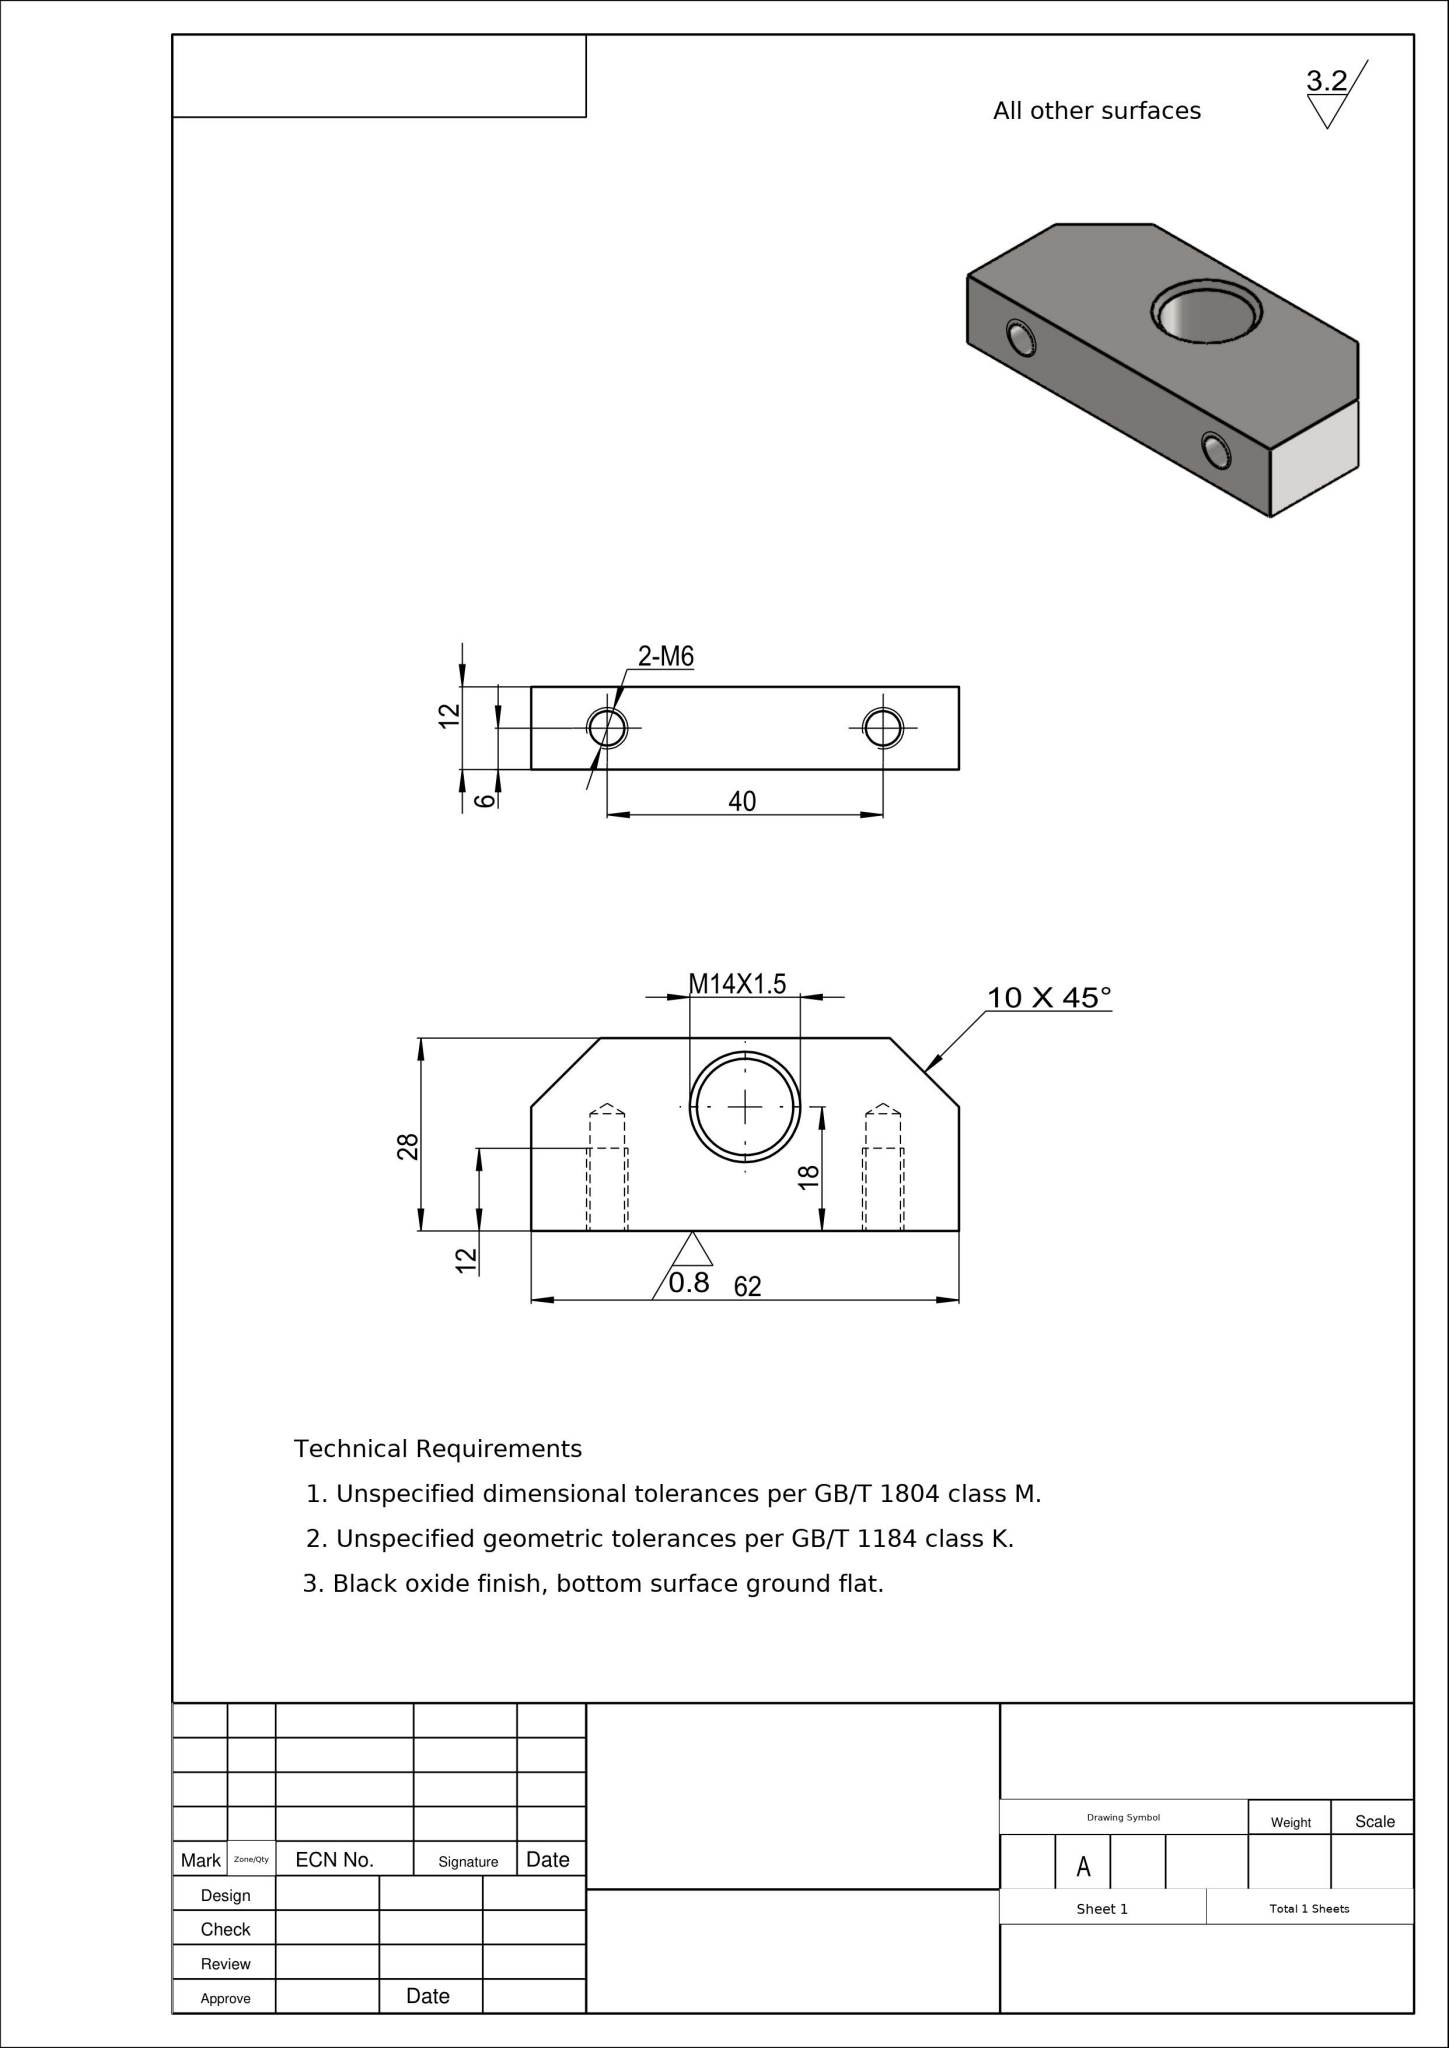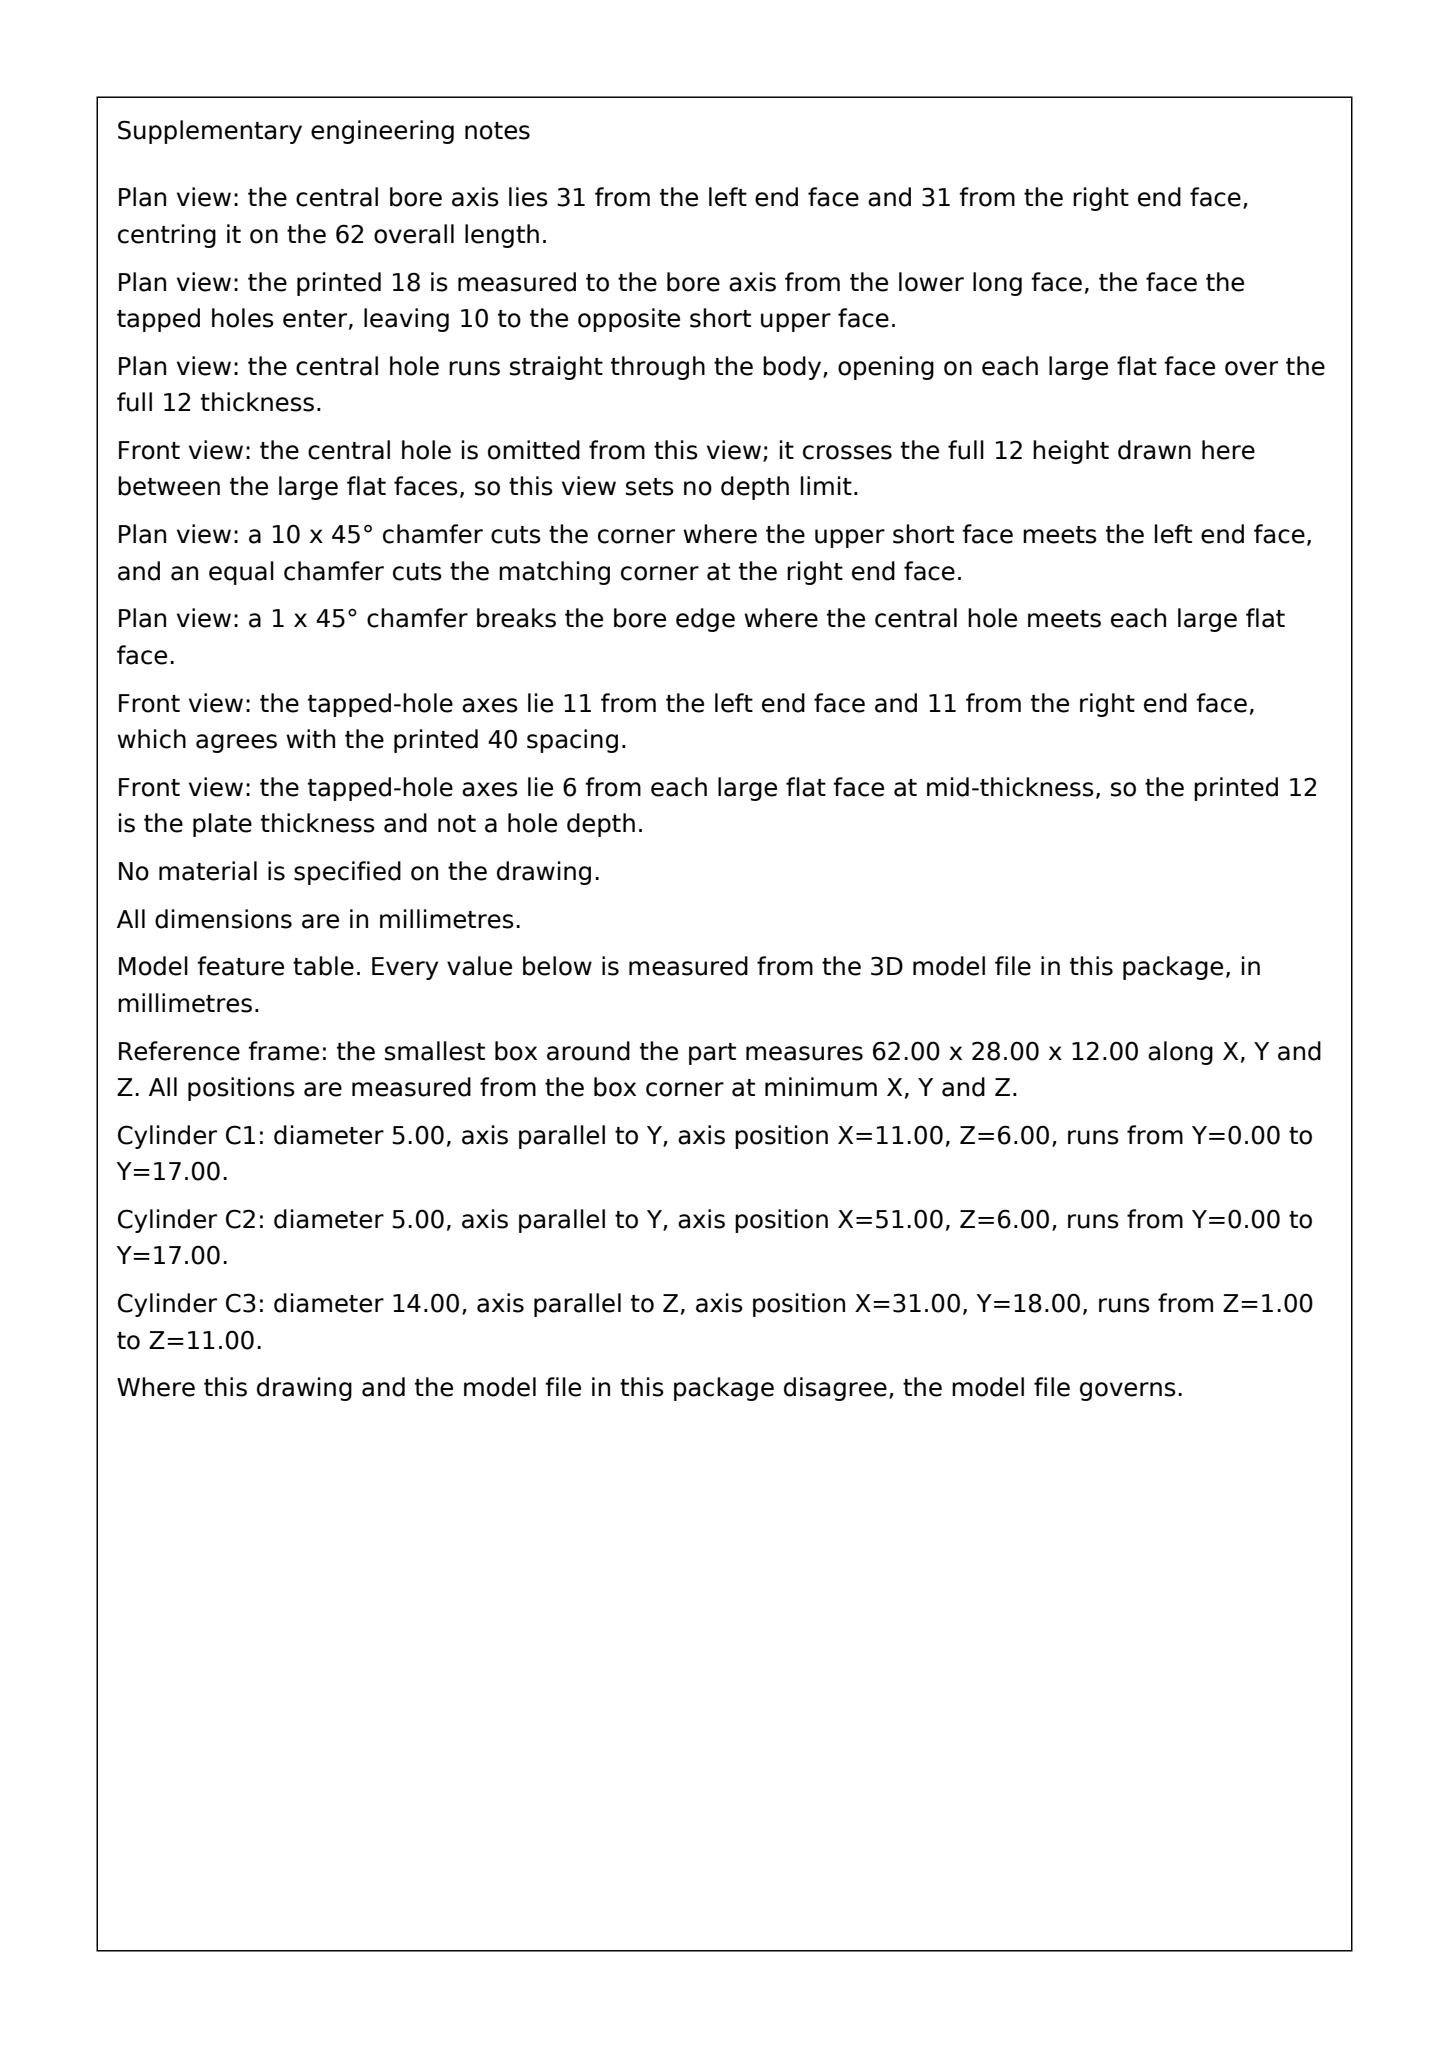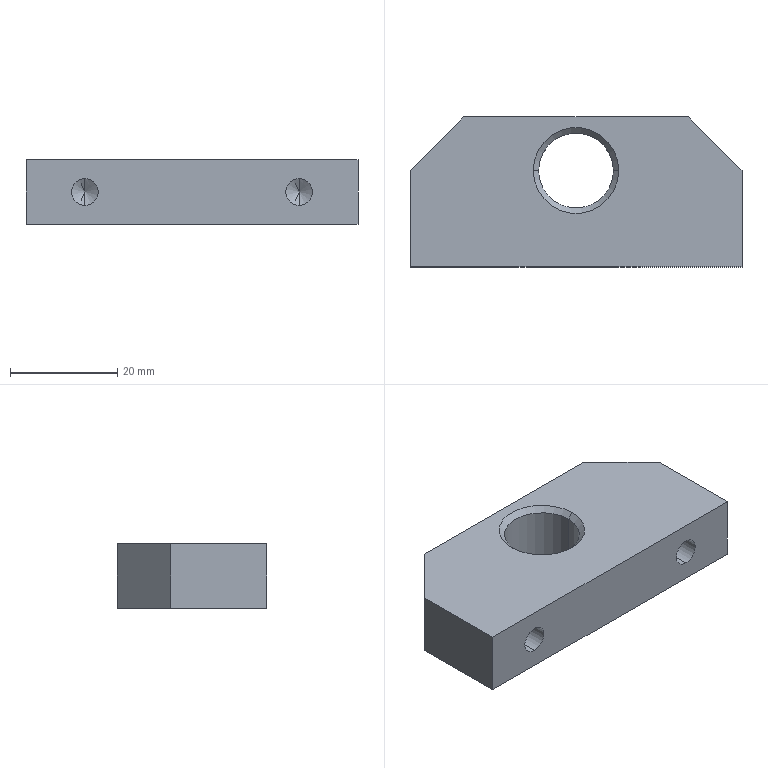Part | SolidWorks | mm | 1 solid | 22 faces | box 62 x 28 x 12 mm | volume 17051 mm3 | cone 8 | plane 8 | cylinder 6 | commonest cylinder face diameters 5 x4 14 x2
Drawing notes:
2-M6 HT 17, DRILL Ø5 HT 17 + 118° PT, FROM SIDE FACE | from the solid: cylinders [5.0,'y',[11.0,null,6.0],17.0] and [5.0,'y',[51.0,null,6.0],17.0]; cones 118.0 ref_dia 5.0
build123d program:
from build123d import *

# Parameters (mm, degrees)
SKETCH1_W             = 62
SKETCH1_H             = 28
BOSS_EXTRUDE1_DEPTH   = 12
M6_TAPPED_HOLE1_D     = 5
M6_TAPPED_HOLE1_DEPTH = 17
M6_TAPPED_HOLE1_TIP   = 1.502
CHAMFER1_SIZE         = 10
SKETCH4_R             = 7
CUT_EXTRUDE1_DEPTH    = 70.08
CHAMFER2_SIZE         = 1


with BuildPart() as part:
    # Sketch1 → Boss-Extrude1 (new body)
    with BuildSketch(Plane.XY):
        with Locations((31, -14)):
            Rectangle(SKETCH1_W, SKETCH1_H)
    extrude(amount=BOSS_EXTRUDE1_DEPTH)

    # M6 Tapped Hole1
    with Locations(Plane.XZ.offset(28)):
        with Locations((11, 6), (51, 6)):
            Hole(M6_TAPPED_HOLE1_D / 2, depth=M6_TAPPED_HOLE1_DEPTH)
            with Locations((0, 0, -(M6_TAPPED_HOLE1_DEPTH + M6_TAPPED_HOLE1_TIP / 2))):  # 118° drill point
                Cone(0, M6_TAPPED_HOLE1_D / 2, M6_TAPPED_HOLE1_TIP, mode=Mode.SUBTRACT)

    # Chamfer1
    chamfer1_edges = [part.edges().sort_by_distance(p)[0] for p in [
        (0, 0, 6),
        (62, 0, 6),
    ]]
    chamfer(chamfer1_edges, length=CHAMFER1_SIZE)

    # Sketch4 → Cut-Extrude1 (cut, through all)
    with BuildSketch(Plane(origin=(0, 0, 0), x_dir=(-1, 0, 0), z_dir=(0, 0, -1))):
        with Locations((-31, -10)):
            Circle(SKETCH4_R)
    extrude(amount=-CUT_EXTRUDE1_DEPTH, mode=Mode.SUBTRACT)

    # Chamfer2
    chamfer2_edges = [part.edges().sort_by_distance(p)[0] for p in [
        (38, -10, 12),
        (38, -10, 0),
    ]]
    chamfer(chamfer2_edges, length=CHAMFER2_SIZE)


solid = part.part
STEP:
#1=CARTESIAN_POINT('',(24.,-10.,11.));
#2=VERTEX_POINT('',#1);
#3=CARTESIAN_POINT('',(38.,-10.,11.));
#4=VERTEX_POINT('',#3);
#5=CARTESIAN_POINT('',(31.,-10.,11.));
#6=DIRECTION('',(0.,0.,1.));
#7=DIRECTION('',(1.,0.,0.));
#8=AXIS2_PLACEMENT_3D('',#5,#6,#7);
#9=CIRCLE('',#8,7.);
#10=EDGE_CURVE('',#2,#4,#9,.T.);
#11=ORIENTED_EDGE('',*,*,#10,.F.);
#12=CARTESIAN_POINT('',(23.,-10.,12.));
#13=VERTEX_POINT('',#12);
#14=CARTESIAN_POINT('',(23.,-10.,12.));
#15=DIRECTION('',(-0.7071,0.,0.7071));
#16=VECTOR('',#15,1000.);
#17=LINE('',#14,#16);
#18=EDGE_CURVE('',#2,#13,#17,.T.);
#19=ORIENTED_EDGE('',*,*,#18,.T.);
#20=CARTESIAN_POINT('',(39.,-10.,12.));
#21=VERTEX_POINT('',#20);
#22=CARTESIAN_POINT('',(31.,-10.,12.));
#23=DIRECTION('',(0.,0.,-1.));
#24=DIRECTION('',(1.,0.,0.));
#25=AXIS2_PLACEMENT_3D('',#22,#23,#24);
#26=CIRCLE('',#25,8.);
#27=EDGE_CURVE('',#21,#13,#26,.T.);
#28=ORIENTED_EDGE('',*,*,#27,.F.);
#29=CARTESIAN_POINT('',(39.,-10.,12.));
#30=DIRECTION('',(0.7071,0.,0.7071));
#31=VECTOR('',#30,1000.);
#32=LINE('',#29,#31);
#33=EDGE_CURVE('',#4,#21,#32,.T.);
#34=ORIENTED_EDGE('',*,*,#33,.F.);
#35=EDGE_LOOP('',(#11,#19,#28,#34));
#36=FACE_OUTER_BOUND('',#35,.T.);
#37=CARTESIAN_POINT('',(31.,-10.,12.));
#38=DIRECTION('',(0.,0.,1.));
#39=DIRECTION('',(1.,0.,0.));
#40=AXIS2_PLACEMENT_3D('',#37,#38,#39);
#41=CONICAL_SURFACE('',#40,8.,0.7854);
#42=ADVANCED_FACE('',(#36),#41,.F.);
#43=CARTESIAN_POINT('',(38.,-10.,1.));
#44=VERTEX_POINT('',#43);
#45=CARTESIAN_POINT('',(24.,-10.,1.));
#46=VERTEX_POINT('',#45);
#47=CARTESIAN_POINT('',(31.,-10.,1.));
#48=DIRECTION('',(0.,0.,-1.));
#49=DIRECTION('',(1.,0.,0.));
#50=AXIS2_PLACEMENT_3D('',#47,#48,#49);
#51=CIRCLE('',#50,7.);
#52=EDGE_CURVE('',#44,#46,#51,.T.);
#53=ORIENTED_EDGE('',*,*,#52,.F.);
#54=CARTESIAN_POINT('',(39.,-10.,0.));
#55=VERTEX_POINT('',#54);
#56=CARTESIAN_POINT('',(38.,-10.,1.));
#57=DIRECTION('',(0.7071,0.,-0.7071));
#58=VECTOR('',#57,1000.);
#59=LINE('',#56,#58);
#60=EDGE_CURVE('',#44,#55,#59,.T.);
#61=ORIENTED_EDGE('',*,*,#60,.T.);
#62=CARTESIAN_POINT('',(23.,-10.,0.));
#63=VERTEX_POINT('',#62);
#64=CARTESIAN_POINT('',(31.,-10.,0.));
#65=DIRECTION('',(0.,0.,1.));
#66=DIRECTION('',(1.,0.,0.));
#67=AXIS2_PLACEMENT_3D('',#64,#65,#66);
#68=CIRCLE('',#67,8.);
#69=EDGE_CURVE('',#63,#55,#68,.T.);
#70=ORIENTED_EDGE('',*,*,#69,.F.);
#71=CARTESIAN_POINT('',(24.,-10.,1.));
#72=DIRECTION('',(-0.7071,0.,-0.7071));
#73=VECTOR('',#72,1000.);
#74=LINE('',#71,#73);
#75=EDGE_CURVE('',#46,#63,#74,.T.);
#76=ORIENTED_EDGE('',*,*,#75,.F.);
#77=EDGE_LOOP('',(#53,#61,#70,#76));
#78=FACE_OUTER_BOUND('',#77,.T.);
#79=CARTESIAN_POINT('',(31.,-10.,1.));
#80=DIRECTION('',(0.,0.,-1.));
#81=DIRECTION('',(-1.,0.,0.));
#82=AXIS2_PLACEMENT_3D('',#79,#80,#81);
#83=CONICAL_SURFACE('',#82,7.,0.7854);
#84=ADVANCED_FACE('',(#78),#83,.F.);
#85=ORIENTED_EDGE('',*,*,#10,.T.);
#86=CARTESIAN_POINT('',(38.,-10.,12.));
#87=DIRECTION('',(0.,0.,-1.));
#88=VECTOR('',#87,1000.);
#89=LINE('',#86,#88);
#90=EDGE_CURVE('',#4,#44,#89,.T.);
#91=ORIENTED_EDGE('',*,*,#90,.T.);
#92=ORIENTED_EDGE('',*,*,#52,.T.);
#93=CARTESIAN_POINT('',(24.,-10.,12.));
#94=DIRECTION('',(0.,0.,-1.));
#95=VECTOR('',#94,1000.);
#96=LINE('',#93,#95);
#97=EDGE_CURVE('',#2,#46,#96,.T.);
#98=ORIENTED_EDGE('',*,*,#97,.F.);
#99=EDGE_LOOP('',(#85,#91,#92,#98));
#100=FACE_OUTER_BOUND('',#99,.T.);
#101=CARTESIAN_POINT('',(31.,-10.,12.));
#102=DIRECTION('',(0.,0.,-1.));
#103=DIRECTION('',(-1.,0.,0.));
#104=AXIS2_PLACEMENT_3D('',#101,#102,#103);
#105=CYLINDRICAL_SURFACE('',#104,7.);
#106=ADVANCED_FACE('',(#100),#105,.F.);
#107=CARTESIAN_POINT('',(11.,-11.,8.5));
#108=VERTEX_POINT('',#107);
#109=CARTESIAN_POINT('',(11.,-11.,3.5));
#110=VERTEX_POINT('',#109);
#111=CARTESIAN_POINT('',(11.,-11.,6.));
#112=DIRECTION('',(0.,-1.,0.));
#113=DIRECTION('',(0.,0.,-1.));
#114=AXIS2_PLACEMENT_3D('',#111,#112,#113);
#115=CIRCLE('',#114,2.5);
#116=EDGE_CURVE('',#108,#110,#115,.T.);
#117=ORIENTED_EDGE('',*,*,#116,.F.);
#118=CARTESIAN_POINT('',(11.,-28.,8.5));
#119=VERTEX_POINT('',#118);
#120=CARTESIAN_POINT('',(11.,-28.,8.5));
#121=DIRECTION('',(0.,-1.,0.));
#122=VECTOR('',#121,1000.);
#123=LINE('',#120,#122);
#124=EDGE_CURVE('',#108,#119,#123,.T.);
#125=ORIENTED_EDGE('',*,*,#124,.T.);
#126=CARTESIAN_POINT('',(11.,-28.,3.5));
#127=VERTEX_POINT('',#126);
#128=CARTESIAN_POINT('',(11.,-28.,6.));
#129=DIRECTION('',(0.,-1.,0.));
#130=DIRECTION('',(0.,0.,-1.));
#131=AXIS2_PLACEMENT_3D('',#128,#129,#130);
#132=CIRCLE('',#131,2.5);
#133=EDGE_CURVE('',#119,#127,#132,.T.);
#134=ORIENTED_EDGE('',*,*,#133,.T.);
#135=CARTESIAN_POINT('',(11.,-28.,3.5));
#136=DIRECTION('',(0.,-1.,0.));
#137=VECTOR('',#136,1000.);
#138=LINE('',#135,#137);
#139=EDGE_CURVE('',#110,#127,#138,.T.);
#140=ORIENTED_EDGE('',*,*,#139,.F.);
#141=EDGE_LOOP('',(#117,#125,#134,#140));
#142=FACE_OUTER_BOUND('',#141,.T.);
#143=CARTESIAN_POINT('',(11.,-28.,6.));
#144=DIRECTION('',(0.,-1.,0.));
#145=DIRECTION('',(0.,0.,-1.));
#146=AXIS2_PLACEMENT_3D('',#143,#144,#145);
#147=CYLINDRICAL_SURFACE('',#146,2.5);
#148=ADVANCED_FACE('',(#142),#147,.F.);
#149=CARTESIAN_POINT('',(11.,-9.498,6.));
#150=VERTEX_POINT('',#149);
#151=CARTESIAN_POINT('',(11.,-11.,3.5));
#152=DIRECTION('',(0.,-0.515,-0.8572));
#153=VECTOR('',#152,1000.);
#154=LINE('',#151,#153);
#155=EDGE_CURVE('',#150,#110,#154,.T.);
#156=ORIENTED_EDGE('',*,*,#155,.F.);
#157=CARTESIAN_POINT('',(11.,-11.,8.5));
#158=DIRECTION('',(0.,-0.515,0.8572));
#159=VECTOR('',#158,1000.);
#160=LINE('',#157,#159);
#161=EDGE_CURVE('',#150,#108,#160,.T.);
#162=ORIENTED_EDGE('',*,*,#161,.T.);
#163=ORIENTED_EDGE('',*,*,#116,.T.);
#164=EDGE_LOOP('',(#156,#162,#163));
#165=FACE_OUTER_BOUND('',#164,.T.);
#166=CARTESIAN_POINT('',(11.,-11.,6.));
#167=DIRECTION('',(0.,-1.,0.));
#168=DIRECTION('',(0.,0.,-1.));
#169=AXIS2_PLACEMENT_3D('',#166,#167,#168);
#170=CONICAL_SURFACE('',#169,2.5,1.03);
#171=ADVANCED_FACE('',(#165),#170,.F.);
#172=CARTESIAN_POINT('',(51.,-11.,8.5));
#173=VERTEX_POINT('',#172);
#174=CARTESIAN_POINT('',(51.,-11.,3.5));
#175=VERTEX_POINT('',#174);
#176=CARTESIAN_POINT('',(51.,-11.,6.));
#177=DIRECTION('',(0.,-1.,0.));
#178=DIRECTION('',(0.,0.,-1.));
#179=AXIS2_PLACEMENT_3D('',#176,#177,#178);
#180=CIRCLE('',#179,2.5);
#181=EDGE_CURVE('',#173,#175,#180,.T.);
#182=ORIENTED_EDGE('',*,*,#181,.F.);
#183=CARTESIAN_POINT('',(51.,-28.,8.5));
#184=VERTEX_POINT('',#183);
#185=CARTESIAN_POINT('',(51.,-28.,8.5));
#186=DIRECTION('',(0.,-1.,0.));
#187=VECTOR('',#186,1000.);
#188=LINE('',#185,#187);
#189=EDGE_CURVE('',#173,#184,#188,.T.);
#190=ORIENTED_EDGE('',*,*,#189,.T.);
#191=CARTESIAN_POINT('',(51.,-28.,3.5));
#192=VERTEX_POINT('',#191);
#193=CARTESIAN_POINT('',(51.,-28.,6.));
#194=DIRECTION('',(0.,-1.,0.));
#195=DIRECTION('',(0.,0.,-1.));
#196=AXIS2_PLACEMENT_3D('',#193,#194,#195);
#197=CIRCLE('',#196,2.5);
#198=EDGE_CURVE('',#184,#192,#197,.T.);
#199=ORIENTED_EDGE('',*,*,#198,.T.);
#200=CARTESIAN_POINT('',(51.,-28.,3.5));
#201=DIRECTION('',(0.,-1.,0.));
#202=VECTOR('',#201,1000.);
#203=LINE('',#200,#202);
#204=EDGE_CURVE('',#175,#192,#203,.T.);
#205=ORIENTED_EDGE('',*,*,#204,.F.);
#206=EDGE_LOOP('',(#182,#190,#199,#205));
#207=FACE_OUTER_BOUND('',#206,.T.);
#208=CARTESIAN_POINT('',(51.,-28.,6.));
#209=DIRECTION('',(0.,-1.,0.));
#210=DIRECTION('',(0.,0.,-1.));
#211=AXIS2_PLACEMENT_3D('',#208,#209,#210);
#212=CYLINDRICAL_SURFACE('',#211,2.5);
#213=ADVANCED_FACE('',(#207),#212,.F.);
#214=CARTESIAN_POINT('',(51.,-9.498,6.));
#215=VERTEX_POINT('',#214);
#216=CARTESIAN_POINT('',(51.,-11.,3.5));
#217=DIRECTION('',(0.,-0.515,-0.8572));
#218=VECTOR('',#217,1000.);
#219=LINE('',#216,#218);
#220=EDGE_CURVE('',#215,#175,#219,.T.);
#221=ORIENTED_EDGE('',*,*,#220,.F.);
#222=CARTESIAN_POINT('',(51.,-11.,8.5));
#223=DIRECTION('',(0.,-0.515,0.8572));
#224=VECTOR('',#223,1000.);
#225=LINE('',#222,#224);
#226=EDGE_CURVE('',#215,#173,#225,.T.);
#227=ORIENTED_EDGE('',*,*,#226,.T.);
#228=ORIENTED_EDGE('',*,*,#181,.T.);
#229=EDGE_LOOP('',(#221,#227,#228));
#230=FACE_OUTER_BOUND('',#229,.T.);
#231=CARTESIAN_POINT('',(51.,-11.,6.));
#232=DIRECTION('',(0.,-1.,0.));
#233=DIRECTION('',(0.,0.,-1.));
#234=AXIS2_PLACEMENT_3D('',#231,#232,#233);
#235=CONICAL_SURFACE('',#234,2.5,1.03);
#236=ADVANCED_FACE('',(#230),#235,.F.);
#237=CARTESIAN_POINT('',(0.,-10.,12.));
#238=VERTEX_POINT('',#237);
#239=CARTESIAN_POINT('',(0.,-28.,12.));
#240=VERTEX_POINT('',#239);
#241=CARTESIAN_POINT('',(0.,0.,12.));
#242=DIRECTION('',(0.,-1.,0.));
#243=VECTOR('',#242,1000.);
#244=LINE('',#241,#243);
#245=EDGE_CURVE('',#238,#240,#244,.T.);
#246=ORIENTED_EDGE('',*,*,#245,.F.);
#247=CARTESIAN_POINT('',(0.,-10.,0.));
#248=VERTEX_POINT('',#247);
#249=CARTESIAN_POINT('',(0.,-10.,12.));
#250=DIRECTION('',(0.,0.,-1.));
#251=VECTOR('',#250,1000.);
#252=LINE('',#249,#251);
#253=EDGE_CURVE('',#238,#248,#252,.T.);
#254=ORIENTED_EDGE('',*,*,#253,.T.);
#255=CARTESIAN_POINT('',(0.,-28.,0.));
#256=VERTEX_POINT('',#255);
#257=CARTESIAN_POINT('',(0.,0.,0.));
#258=DIRECTION('',(0.,-1.,0.));
#259=VECTOR('',#258,1000.);
#260=LINE('',#257,#259);
#261=EDGE_CURVE('',#248,#256,#260,.T.);
#262=ORIENTED_EDGE('',*,*,#261,.T.);
#263=CARTESIAN_POINT('',(0.,-28.,12.));
#264=DIRECTION('',(0.,0.,-1.));
#265=VECTOR('',#264,1000.);
#266=LINE('',#263,#265);
#267=EDGE_CURVE('',#240,#256,#266,.T.);
#268=ORIENTED_EDGE('',*,*,#267,.F.);
#269=EDGE_LOOP('',(#246,#254,#262,#268));
#270=FACE_OUTER_BOUND('',#269,.T.);
#271=CARTESIAN_POINT('',(0.,0.,12.));
#272=DIRECTION('',(1.,0.,0.));
#273=DIRECTION('',(-0.,1.,0.));
#274=AXIS2_PLACEMENT_3D('',#271,#272,#273);
#275=PLANE('',#274);
#276=ADVANCED_FACE('',(#270),#275,.F.);
#277=CARTESIAN_POINT('',(11.,-28.,6.));
#278=DIRECTION('',(0.,-1.,0.));
#279=DIRECTION('',(0.,0.,-1.));
#280=AXIS2_PLACEMENT_3D('',#277,#278,#279);
#281=CIRCLE('',#280,2.5);
#282=EDGE_CURVE('',#127,#119,#281,.T.);
#283=ORIENTED_EDGE('',*,*,#282,.F.);
#284=ORIENTED_EDGE('',*,*,#133,.F.);
#285=EDGE_LOOP('',(#283,#284));
#286=FACE_BOUND('',#285,.T.);
#287=CARTESIAN_POINT('',(51.,-28.,6.));
#288=DIRECTION('',(0.,-1.,0.));
#289=DIRECTION('',(0.,0.,-1.));
#290=AXIS2_PLACEMENT_3D('',#287,#288,#289);
#291=CIRCLE('',#290,2.5);
#292=EDGE_CURVE('',#192,#184,#291,.T.);
#293=ORIENTED_EDGE('',*,*,#292,.F.);
#294=ORIENTED_EDGE('',*,*,#198,.F.);
#295=EDGE_LOOP('',(#293,#294));
#296=FACE_BOUND('',#295,.T.);
#297=CARTESIAN_POINT('',(62.,-28.,0.));
#298=VERTEX_POINT('',#297);
#299=CARTESIAN_POINT('',(0.,-28.,0.));
#300=DIRECTION('',(1.,0.,0.));
#301=VECTOR('',#300,1000.);
#302=LINE('',#299,#301);
#303=EDGE_CURVE('',#256,#298,#302,.T.);
#304=ORIENTED_EDGE('',*,*,#303,.T.);
#305=CARTESIAN_POINT('',(62.,-28.,12.));
#306=VERTEX_POINT('',#305);
#307=CARTESIAN_POINT('',(62.,-28.,12.));
#308=DIRECTION('',(0.,0.,-1.));
#309=VECTOR('',#308,1000.);
#310=LINE('',#307,#309);
#311=EDGE_CURVE('',#306,#298,#310,.T.);
#312=ORIENTED_EDGE('',*,*,#311,.F.);
#313=CARTESIAN_POINT('',(0.,-28.,12.));
#314=DIRECTION('',(1.,0.,0.));
#315=VECTOR('',#314,1000.);
#316=LINE('',#313,#315);
#317=EDGE_CURVE('',#240,#306,#316,.T.);
#318=ORIENTED_EDGE('',*,*,#317,.F.);
#319=ORIENTED_EDGE('',*,*,#267,.T.);
#320=EDGE_LOOP('',(#304,#312,#318,#319));
#321=FACE_OUTER_BOUND('',#320,.T.);
#322=CARTESIAN_POINT('',(0.,-28.,12.));
#323=DIRECTION('',(0.,1.,0.));
#324=DIRECTION('',(0.,0.,1.));
#325=AXIS2_PLACEMENT_3D('',#322,#323,#324);
#326=PLANE('',#325);
#327=ADVANCED_FACE('',(#286,#296,#321),#326,.F.);
#328=CARTESIAN_POINT('',(62.,-10.,0.));
#329=VERTEX_POINT('',#328);
#330=CARTESIAN_POINT('',(62.,0.,0.));
#331=DIRECTION('',(0.,1.,0.));
#332=VECTOR('',#331,1000.);
#333=LINE('',#330,#332);
#334=EDGE_CURVE('',#298,#329,#333,.T.);
#335=ORIENTED_EDGE('',*,*,#334,.T.);
#336=CARTESIAN_POINT('',(62.,-10.,12.));
#337=VERTEX_POINT('',#336);
#338=CARTESIAN_POINT('',(62.,-10.,12.));
#339=DIRECTION('',(0.,0.,1.));
#340=VECTOR('',#339,1000.);
#341=LINE('',#338,#340);
#342=EDGE_CURVE('',#329,#337,#341,.T.);
#343=ORIENTED_EDGE('',*,*,#342,.T.);
#344=CARTESIAN_POINT('',(62.,0.,12.));
#345=DIRECTION('',(0.,1.,0.));
#346=VECTOR('',#345,1000.);
#347=LINE('',#344,#346);
#348=EDGE_CURVE('',#306,#337,#347,.T.);
#349=ORIENTED_EDGE('',*,*,#348,.F.);
#350=ORIENTED_EDGE('',*,*,#311,.T.);
#351=EDGE_LOOP('',(#335,#343,#349,#350));
#352=FACE_OUTER_BOUND('',#351,.T.);
#353=CARTESIAN_POINT('',(62.,0.,12.));
#354=DIRECTION('',(-1.,0.,0.));
#355=DIRECTION('',(0.,0.,1.));
#356=AXIS2_PLACEMENT_3D('',#353,#354,#355);
#357=PLANE('',#356);
#358=ADVANCED_FACE('',(#352),#357,.F.);
#359=CARTESIAN_POINT('',(52.,0.,0.));
#360=VERTEX_POINT('',#359);
#361=CARTESIAN_POINT('',(10.,0.,0.));
#362=VERTEX_POINT('',#361);
#363=CARTESIAN_POINT('',(0.,0.,0.));
#364=DIRECTION('',(-1.,0.,0.));
#365=VECTOR('',#364,1000.);
#366=LINE('',#363,#365);
#367=EDGE_CURVE('',#360,#362,#366,.T.);
#368=ORIENTED_EDGE('',*,*,#367,.T.);
#369=CARTESIAN_POINT('',(10.,0.,12.));
#370=VERTEX_POINT('',#369);
#371=CARTESIAN_POINT('',(10.,0.,12.));
#372=DIRECTION('',(0.,0.,1.));
#373=VECTOR('',#372,1000.);
#374=LINE('',#371,#373);
#375=EDGE_CURVE('',#362,#370,#374,.T.);
#376=ORIENTED_EDGE('',*,*,#375,.T.);
#377=CARTESIAN_POINT('',(52.,0.,12.));
#378=VERTEX_POINT('',#377);
#379=CARTESIAN_POINT('',(0.,0.,12.));
#380=DIRECTION('',(-1.,0.,0.));
#381=VECTOR('',#380,1000.);
#382=LINE('',#379,#381);
#383=EDGE_CURVE('',#378,#370,#382,.T.);
#384=ORIENTED_EDGE('',*,*,#383,.F.);
#385=CARTESIAN_POINT('',(52.,0.,12.));
#386=DIRECTION('',(0.,0.,-1.));
#387=VECTOR('',#386,1000.);
#388=LINE('',#385,#387);
#389=EDGE_CURVE('',#378,#360,#388,.T.);
#390=ORIENTED_EDGE('',*,*,#389,.T.);
#391=EDGE_LOOP('',(#368,#376,#384,#390));
#392=FACE_OUTER_BOUND('',#391,.T.);
#393=CARTESIAN_POINT('',(0.,0.,12.));
#394=DIRECTION('',(0.,-1.,0.));
#395=DIRECTION('',(0.,0.,-1.));
#396=AXIS2_PLACEMENT_3D('',#393,#394,#395);
#397=PLANE('',#396);
#398=ADVANCED_FACE('',(#392),#397,.F.);
#399=ORIENTED_EDGE('',*,*,#27,.T.);
#400=CARTESIAN_POINT('',(31.,-10.,12.));
#401=DIRECTION('',(0.,0.,-1.));
#402=DIRECTION('',(1.,0.,0.));
#403=AXIS2_PLACEMENT_3D('',#400,#401,#402);
#404=CIRCLE('',#403,8.);
#405=EDGE_CURVE('',#13,#21,#404,.T.);
#406=ORIENTED_EDGE('',*,*,#405,.T.);
#407=EDGE_LOOP('',(#399,#406));
#408=FACE_BOUND('',#407,.T.);
#409=ORIENTED_EDGE('',*,*,#383,.T.);
#410=CARTESIAN_POINT('',(-9.,-19.,12.));
#411=DIRECTION('',(-0.7071,-0.7071,0.));
#412=VECTOR('',#411,1000.);
#413=LINE('',#410,#412);
#414=EDGE_CURVE('',#370,#238,#413,.T.);
#415=ORIENTED_EDGE('',*,*,#414,.T.);
#416=ORIENTED_EDGE('',*,*,#245,.T.);
#417=ORIENTED_EDGE('',*,*,#317,.T.);
#418=ORIENTED_EDGE('',*,*,#348,.T.);
#419=CARTESIAN_POINT('',(40.,12.,12.));
#420=DIRECTION('',(-0.7071,0.7071,0.));
#421=VECTOR('',#420,1000.);
#422=LINE('',#419,#421);
#423=EDGE_CURVE('',#337,#378,#422,.T.);
#424=ORIENTED_EDGE('',*,*,#423,.T.);
#425=EDGE_LOOP('',(#409,#415,#416,#417,#418,#424));
#426=FACE_OUTER_BOUND('',#425,.T.);
#427=CARTESIAN_POINT('',(0.,-28.,12.));
#428=DIRECTION('',(0.,0.,1.));
#429=DIRECTION('',(1.,0.,0.));
#430=AXIS2_PLACEMENT_3D('',#427,#428,#429);
#431=PLANE('',#430);
#432=ADVANCED_FACE('',(#408,#426),#431,.T.);
#433=ORIENTED_EDGE('',*,*,#69,.T.);
#434=CARTESIAN_POINT('',(31.,-10.,0.));
#435=DIRECTION('',(0.,0.,1.));
#436=DIRECTION('',(1.,0.,0.));
#437=AXIS2_PLACEMENT_3D('',#434,#435,#436);
#438=CIRCLE('',#437,8.);
#439=EDGE_CURVE('',#55,#63,#438,.T.);
#440=ORIENTED_EDGE('',*,*,#439,.T.);
#441=EDGE_LOOP('',(#433,#440));
#442=FACE_BOUND('',#441,.T.);
#443=ORIENTED_EDGE('',*,*,#261,.F.);
#444=CARTESIAN_POINT('',(0.,-10.,0.));
#445=DIRECTION('',(0.7071,0.7071,0.));
#446=VECTOR('',#445,1000.);
#447=LINE('',#444,#446);
#448=EDGE_CURVE('',#248,#362,#447,.T.);
#449=ORIENTED_EDGE('',*,*,#448,.T.);
#450=ORIENTED_EDGE('',*,*,#367,.F.);
#451=CARTESIAN_POINT('',(52.,0.,0.));
#452=DIRECTION('',(0.7071,-0.7071,0.));
#453=VECTOR('',#452,1000.);
#454=LINE('',#451,#453);
#455=EDGE_CURVE('',#360,#329,#454,.T.);
#456=ORIENTED_EDGE('',*,*,#455,.T.);
#457=ORIENTED_EDGE('',*,*,#334,.F.);
#458=ORIENTED_EDGE('',*,*,#303,.F.);
#459=EDGE_LOOP('',(#443,#449,#450,#456,#457,#458));
#460=FACE_OUTER_BOUND('',#459,.T.);
#461=CARTESIAN_POINT('',(0.,-28.,0.));
#462=DIRECTION('',(0.,0.,1.));
#463=DIRECTION('',(1.,0.,0.));
#464=AXIS2_PLACEMENT_3D('',#461,#462,#463);
#465=PLANE('',#464);
#466=ADVANCED_FACE('',(#442,#460),#465,.F.);
#467=ORIENTED_EDGE('',*,*,#226,.F.);
#468=ORIENTED_EDGE('',*,*,#220,.T.);
#469=CARTESIAN_POINT('',(51.,-11.,6.));
#470=DIRECTION('',(0.,-1.,0.));
#471=DIRECTION('',(0.,0.,-1.));
#472=AXIS2_PLACEMENT_3D('',#469,#470,#471);
#473=CIRCLE('',#472,2.5);
#474=EDGE_CURVE('',#175,#173,#473,.T.);
#475=ORIENTED_EDGE('',*,*,#474,.T.);
#476=EDGE_LOOP('',(#467,#468,#475));
#477=FACE_OUTER_BOUND('',#476,.T.);
#478=CARTESIAN_POINT('',(51.,-11.,6.));
#479=DIRECTION('',(0.,-1.,0.));
#480=DIRECTION('',(0.,0.,-1.));
#481=AXIS2_PLACEMENT_3D('',#478,#479,#480);
#482=CONICAL_SURFACE('',#481,2.5,1.03);
#483=ADVANCED_FACE('',(#477),#482,.F.);
#484=ORIENTED_EDGE('',*,*,#189,.F.);
#485=ORIENTED_EDGE('',*,*,#474,.F.);
#486=ORIENTED_EDGE('',*,*,#204,.T.);
#487=ORIENTED_EDGE('',*,*,#292,.T.);
#488=EDGE_LOOP('',(#484,#485,#486,#487));
#489=FACE_OUTER_BOUND('',#488,.T.);
#490=CARTESIAN_POINT('',(51.,-28.,6.));
#491=DIRECTION('',(0.,-1.,0.));
#492=DIRECTION('',(0.,0.,-1.));
#493=AXIS2_PLACEMENT_3D('',#490,#491,#492);
#494=CYLINDRICAL_SURFACE('',#493,2.5);
#495=ADVANCED_FACE('',(#489),#494,.F.);
#496=ORIENTED_EDGE('',*,*,#161,.F.);
#497=ORIENTED_EDGE('',*,*,#155,.T.);
#498=CARTESIAN_POINT('',(11.,-11.,6.));
#499=DIRECTION('',(0.,-1.,0.));
#500=DIRECTION('',(0.,0.,-1.));
#501=AXIS2_PLACEMENT_3D('',#498,#499,#500);
#502=CIRCLE('',#501,2.5);
#503=EDGE_CURVE('',#110,#108,#502,.T.);
#504=ORIENTED_EDGE('',*,*,#503,.T.);
#505=EDGE_LOOP('',(#496,#497,#504));
#506=FACE_OUTER_BOUND('',#505,.T.);
#507=CARTESIAN_POINT('',(11.,-11.,6.));
#508=DIRECTION('',(0.,-1.,0.));
#509=DIRECTION('',(0.,0.,-1.));
#510=AXIS2_PLACEMENT_3D('',#507,#508,#509);
#511=CONICAL_SURFACE('',#510,2.5,1.03);
#512=ADVANCED_FACE('',(#506),#511,.F.);
#513=ORIENTED_EDGE('',*,*,#124,.F.);
#514=ORIENTED_EDGE('',*,*,#503,.F.);
#515=ORIENTED_EDGE('',*,*,#139,.T.);
#516=ORIENTED_EDGE('',*,*,#282,.T.);
#517=EDGE_LOOP('',(#513,#514,#515,#516));
#518=FACE_OUTER_BOUND('',#517,.T.);
#519=CARTESIAN_POINT('',(11.,-28.,6.));
#520=DIRECTION('',(0.,-1.,0.));
#521=DIRECTION('',(0.,0.,-1.));
#522=AXIS2_PLACEMENT_3D('',#519,#520,#521);
#523=CYLINDRICAL_SURFACE('',#522,2.5);
#524=ADVANCED_FACE('',(#518),#523,.F.);
#525=ORIENTED_EDGE('',*,*,#414,.F.);
#526=ORIENTED_EDGE('',*,*,#375,.F.);
#527=ORIENTED_EDGE('',*,*,#448,.F.);
#528=ORIENTED_EDGE('',*,*,#253,.F.);
#529=EDGE_LOOP('',(#525,#526,#527,#528));
#530=FACE_OUTER_BOUND('',#529,.T.);
#531=CARTESIAN_POINT('',(0.,-10.,12.));
#532=DIRECTION('',(0.7071,-0.7071,0.));
#533=DIRECTION('',(0.7071,0.7071,0.));
#534=AXIS2_PLACEMENT_3D('',#531,#532,#533);
#535=PLANE('',#534);
#536=ADVANCED_FACE('',(#530),#535,.F.);
#537=ORIENTED_EDGE('',*,*,#423,.F.);
#538=ORIENTED_EDGE('',*,*,#342,.F.);
#539=ORIENTED_EDGE('',*,*,#455,.F.);
#540=ORIENTED_EDGE('',*,*,#389,.F.);
#541=EDGE_LOOP('',(#537,#538,#539,#540));
#542=FACE_OUTER_BOUND('',#541,.T.);
#543=CARTESIAN_POINT('',(52.,0.,12.));
#544=DIRECTION('',(-0.7071,-0.7071,0.));
#545=DIRECTION('',(0.7071,-0.7071,0.));
#546=AXIS2_PLACEMENT_3D('',#543,#544,#545);
#547=PLANE('',#546);
#548=ADVANCED_FACE('',(#542),#547,.F.);
#549=ORIENTED_EDGE('',*,*,#90,.F.);
#550=CARTESIAN_POINT('',(31.,-10.,11.));
#551=DIRECTION('',(0.,0.,1.));
#552=DIRECTION('',(1.,0.,0.));
#553=AXIS2_PLACEMENT_3D('',#550,#551,#552);
#554=CIRCLE('',#553,7.);
#555=EDGE_CURVE('',#4,#2,#554,.T.);
#556=ORIENTED_EDGE('',*,*,#555,.T.);
#557=ORIENTED_EDGE('',*,*,#97,.T.);
#558=CARTESIAN_POINT('',(31.,-10.,1.));
#559=DIRECTION('',(0.,0.,-1.));
#560=DIRECTION('',(1.,0.,0.));
#561=AXIS2_PLACEMENT_3D('',#558,#559,#560);
#562=CIRCLE('',#561,7.);
#563=EDGE_CURVE('',#46,#44,#562,.T.);
#564=ORIENTED_EDGE('',*,*,#563,.T.);
#565=EDGE_LOOP('',(#549,#556,#557,#564));
#566=FACE_OUTER_BOUND('',#565,.T.);
#567=CARTESIAN_POINT('',(31.,-10.,12.));
#568=DIRECTION('',(0.,0.,-1.));
#569=DIRECTION('',(-1.,0.,0.));
#570=AXIS2_PLACEMENT_3D('',#567,#568,#569);
#571=CYLINDRICAL_SURFACE('',#570,7.);
#572=ADVANCED_FACE('',(#566),#571,.F.);
#573=ORIENTED_EDGE('',*,*,#60,.F.);
#574=ORIENTED_EDGE('',*,*,#563,.F.);
#575=ORIENTED_EDGE('',*,*,#75,.T.);
#576=ORIENTED_EDGE('',*,*,#439,.F.);
#577=EDGE_LOOP('',(#573,#574,#575,#576));
#578=FACE_OUTER_BOUND('',#577,.T.);
#579=CARTESIAN_POINT('',(31.,-10.,1.));
#580=DIRECTION('',(0.,0.,-1.));
#581=DIRECTION('',(-1.,0.,0.));
#582=AXIS2_PLACEMENT_3D('',#579,#580,#581);
#583=CONICAL_SURFACE('',#582,7.,0.7854);
#584=ADVANCED_FACE('',(#578),#583,.F.);
#585=ORIENTED_EDGE('',*,*,#18,.F.);
#586=ORIENTED_EDGE('',*,*,#555,.F.);
#587=ORIENTED_EDGE('',*,*,#33,.T.);
#588=ORIENTED_EDGE('',*,*,#405,.F.);
#589=EDGE_LOOP('',(#585,#586,#587,#588));
#590=FACE_OUTER_BOUND('',#589,.T.);
#591=CARTESIAN_POINT('',(31.,-10.,12.));
#592=DIRECTION('',(0.,0.,1.));
#593=DIRECTION('',(1.,0.,0.));
#594=AXIS2_PLACEMENT_3D('',#591,#592,#593);
#595=CONICAL_SURFACE('',#594,8.,0.7854);
#596=ADVANCED_FACE('',(#590),#595,.F.);
#597=CLOSED_SHELL('',(#42,#84,#106,#148,#171,#213,#236,#276,#327,#358,#398,#432,#466,#483,#495,#512,#524,#536,#548,#572,#584,#596));
#598=MANIFOLD_SOLID_BREP('',#597);
#599=CARTESIAN_POINT('',(0.,0.,0.));
#600=DIRECTION('',(0.,0.,1.));
#601=DIRECTION('',(1.,0.,0.));
#602=AXIS2_PLACEMENT_3D('',#599,#600,#601);
#603=(LENGTH_UNIT()NAMED_UNIT(*)SI_UNIT(.MILLI.,.METRE.));
#604=UNCERTAINTY_MEASURE_WITH_UNIT(LENGTH_MEASURE(0.00001),#603,'','');
#605=(NAMED_UNIT(*)PLANE_ANGLE_UNIT()SI_UNIT($,.RADIAN.));
#606=(NAMED_UNIT(*)SI_UNIT($,.STERADIAN.)SOLID_ANGLE_UNIT());
#607=(GEOMETRIC_REPRESENTATION_CONTEXT(3)GLOBAL_UNCERTAINTY_ASSIGNED_CONTEXT((#604))GLOBAL_UNIT_ASSIGNED_CONTEXT((#603,#605,#606))REPRESENTATION_CONTEXT('',''));
#608=ADVANCED_BREP_SHAPE_REPRESENTATION('',(#598,#602),#607);